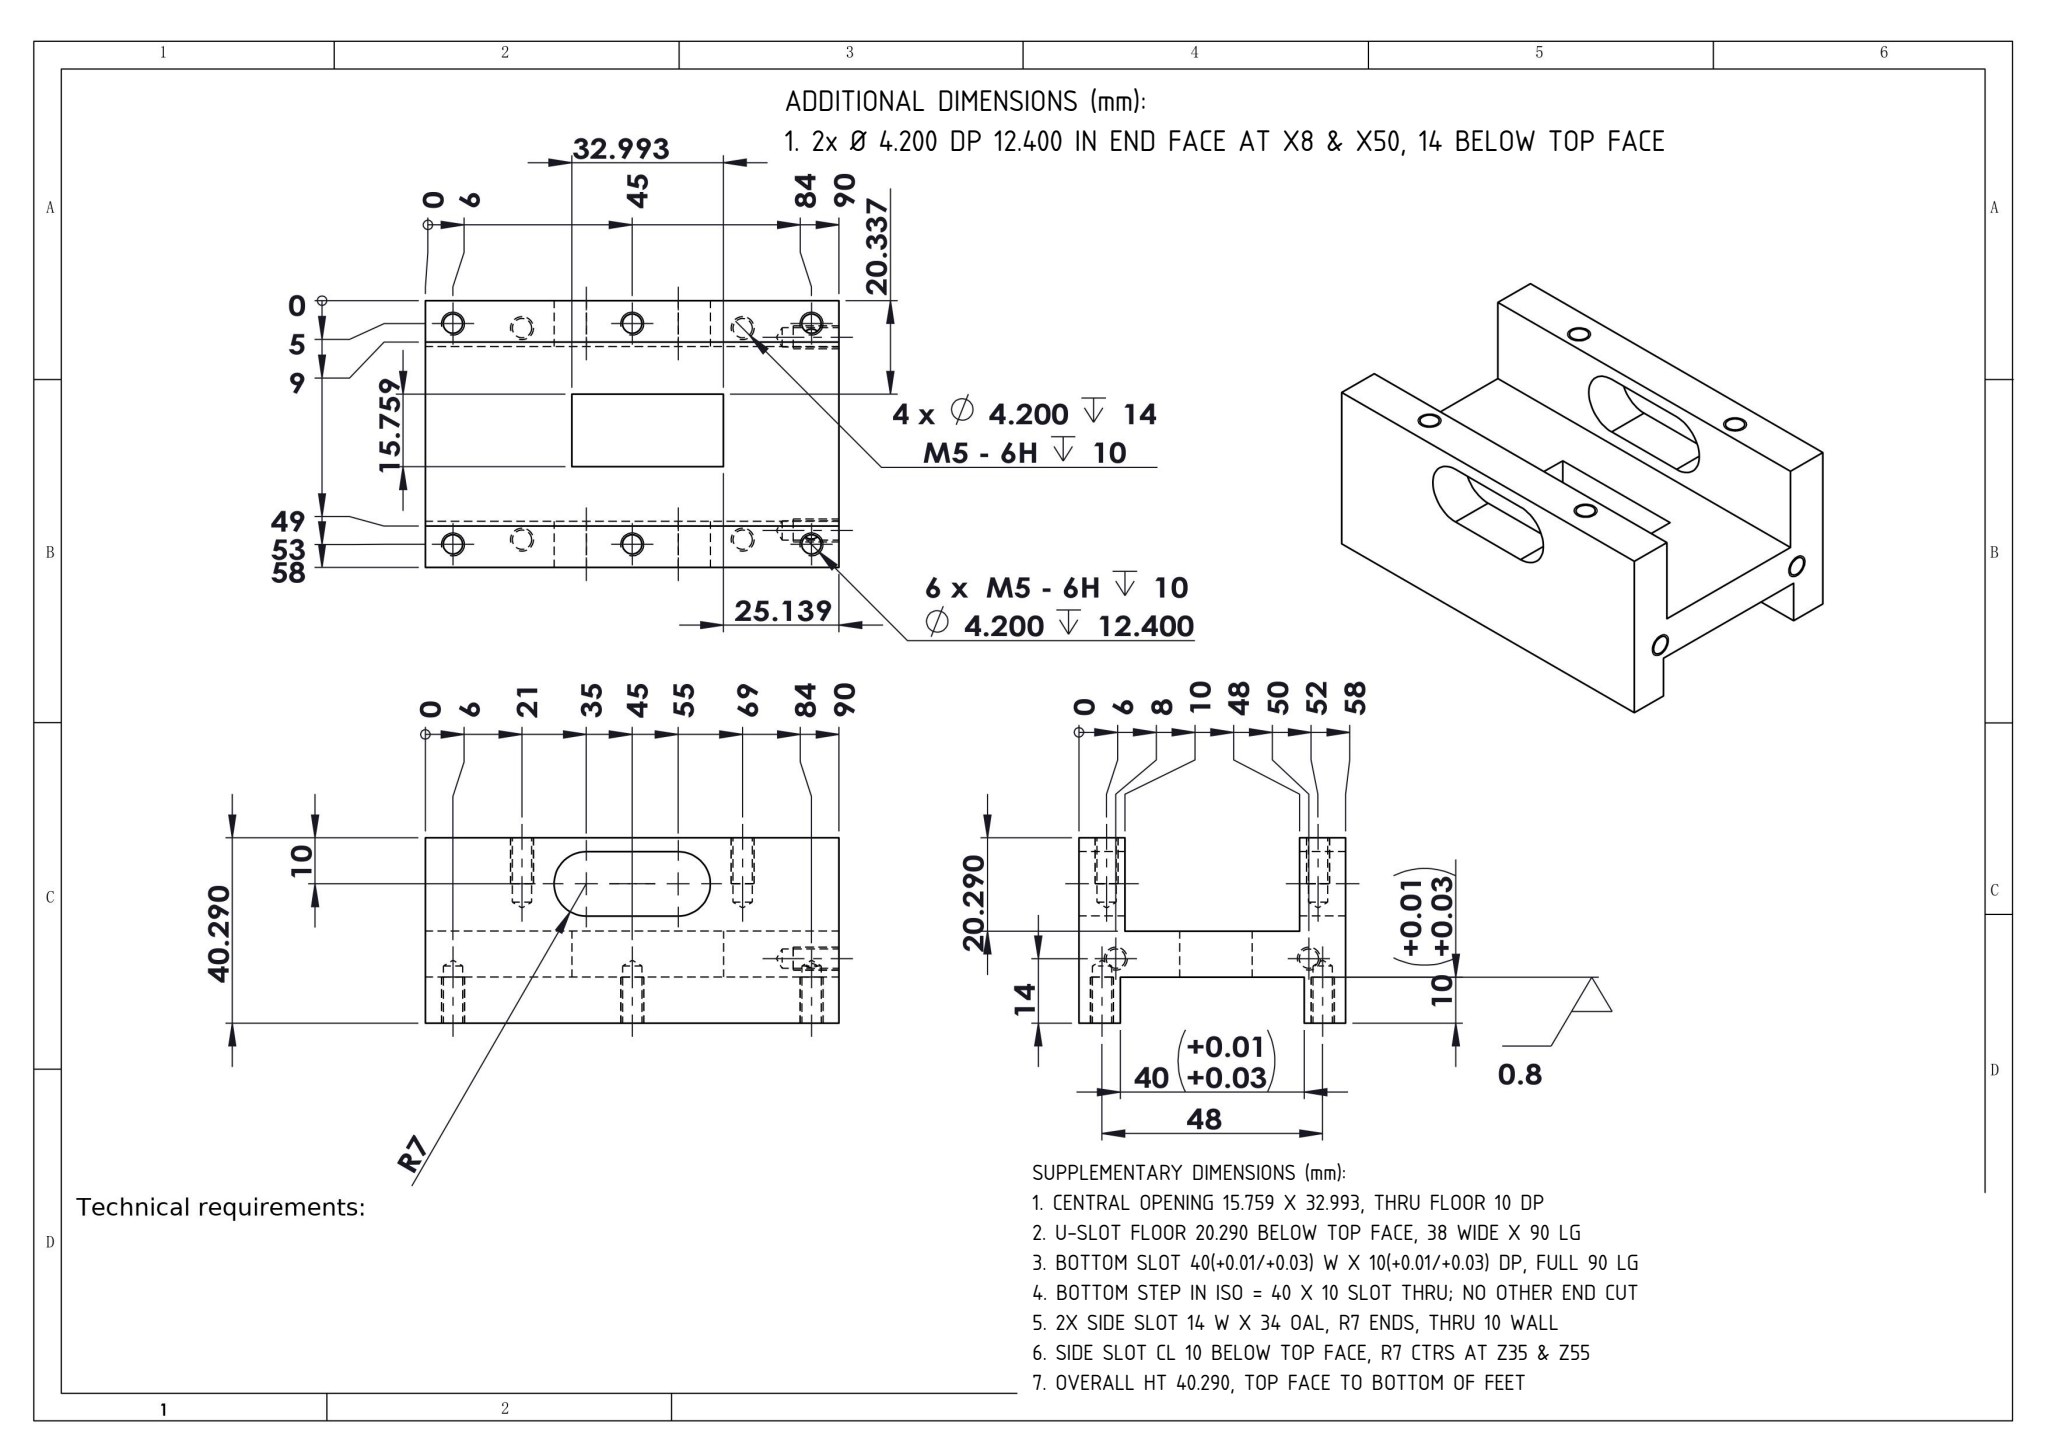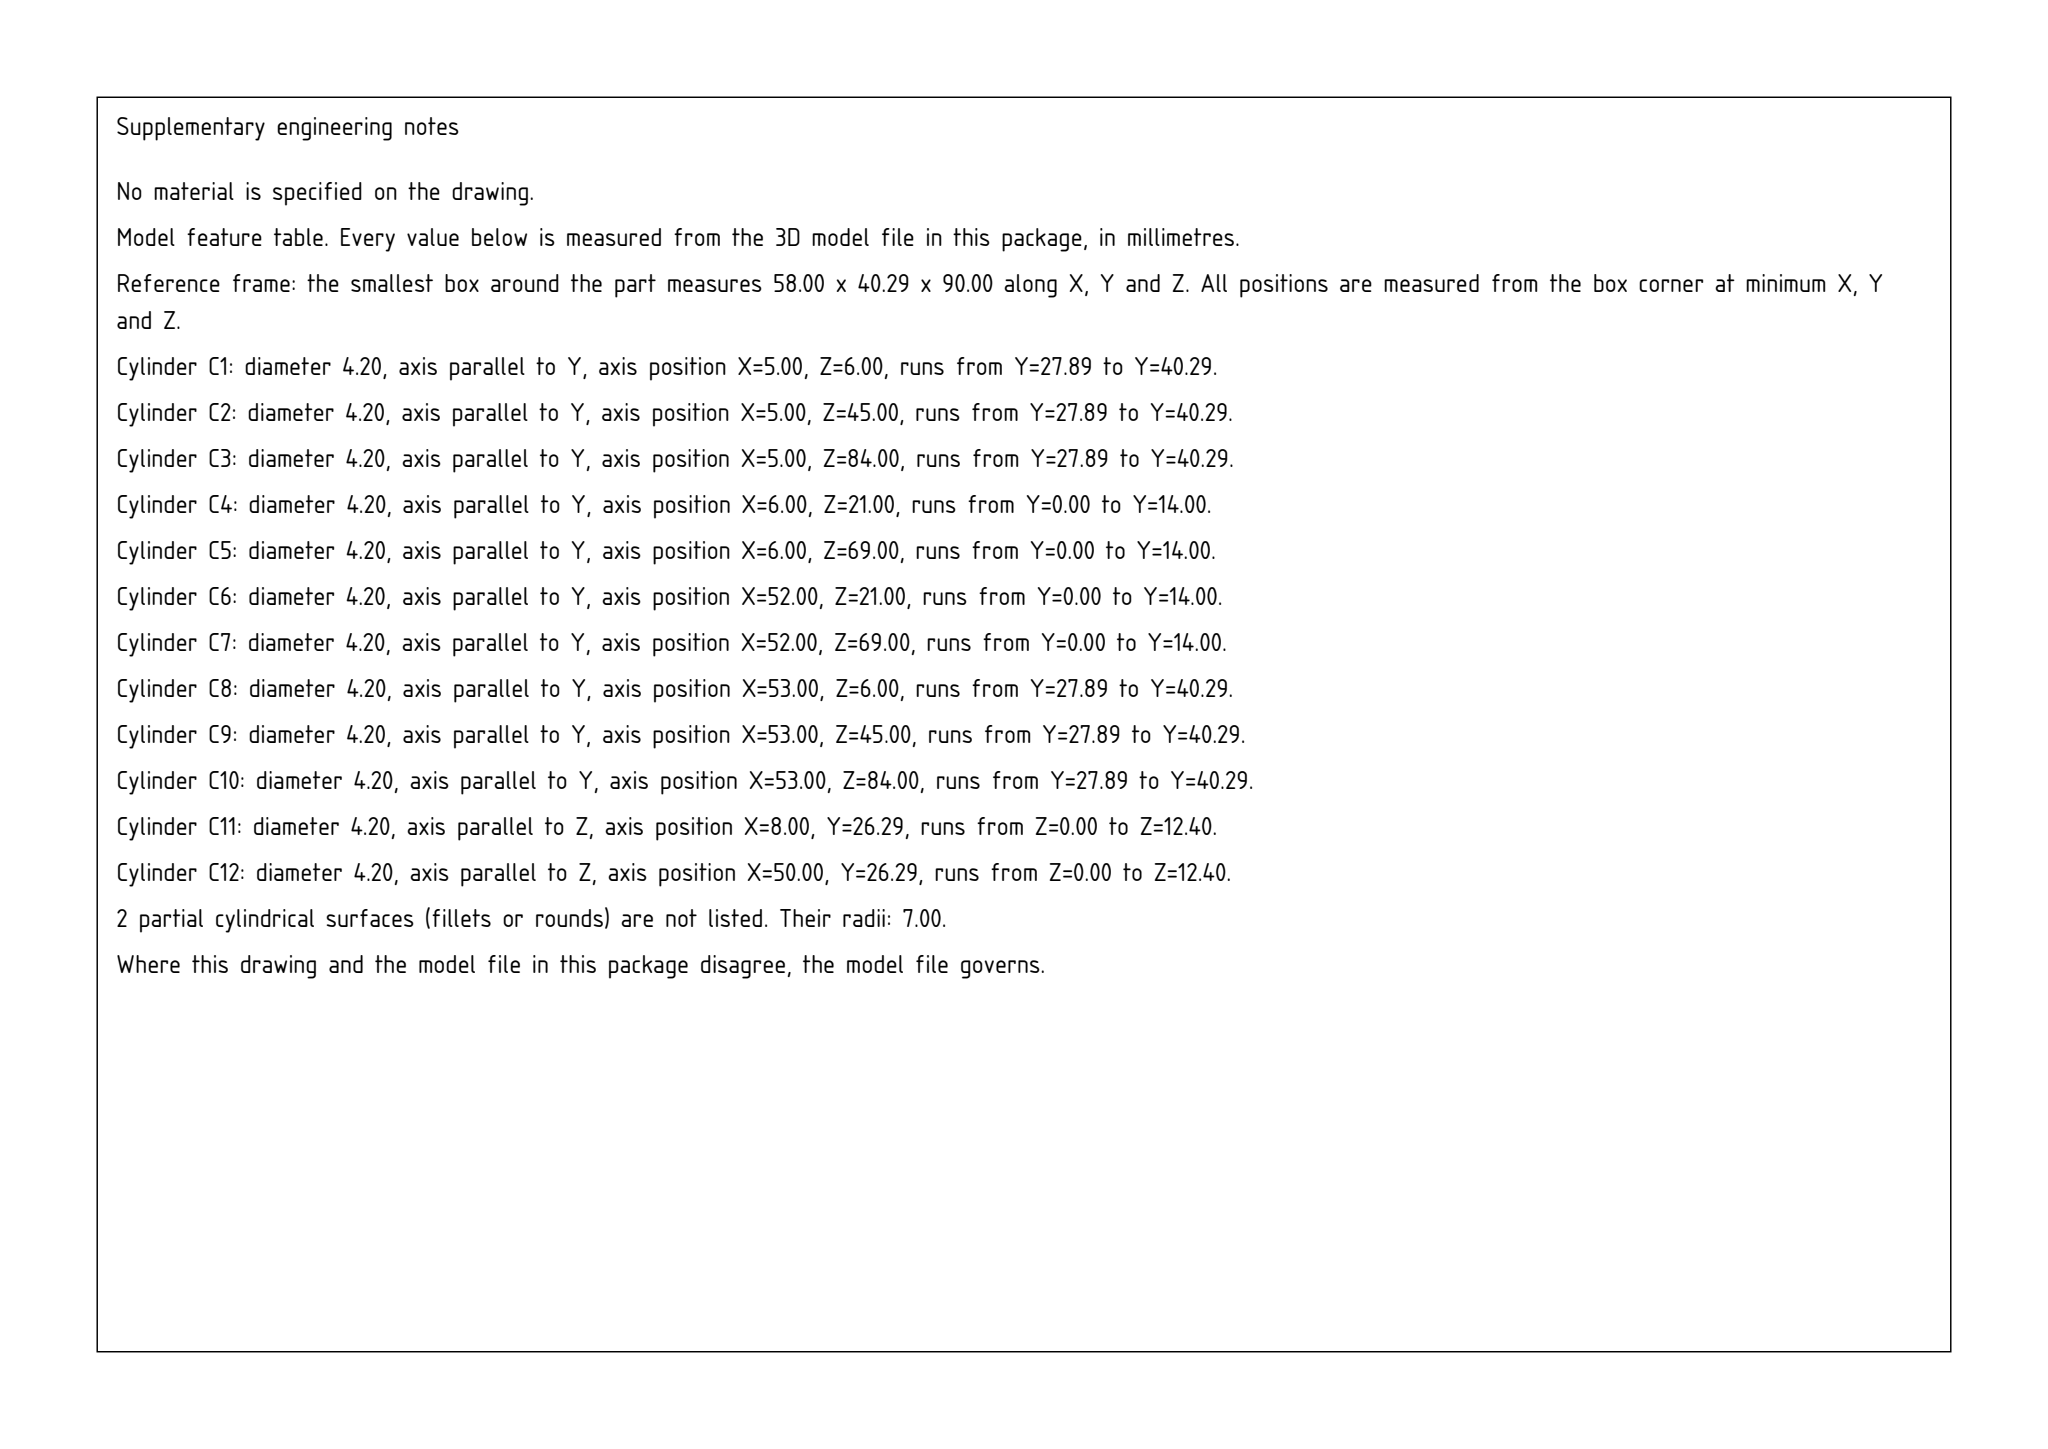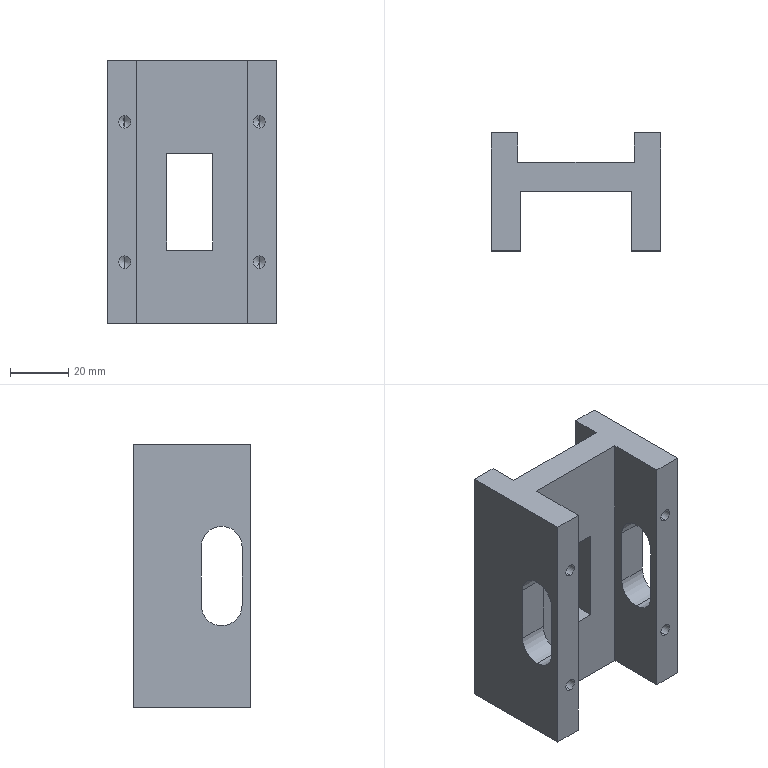Part | SolidWorks | mm | 1 solid | 76 faces | box 58 x 40.29 x 90 mm | volume 88824 mm3 | cylinder 30 | cone 24 | plane 22 | commonest cylinder face diameters 4.2 x24 14 x6
build123d program:
from build123d import *

# Parameters (mm, degrees)
SKETCH1_W             = 58
SKETCH1_H             = 90
BOSS_EXTRUDE1_DEPTH   = 40.29
SKETCH2_W             = 40
SKETCH2_H             = 90
CUT_EXTRUDE1_DEPTH    = 10
M5_TAPPED_HOLE1_D     = 4.2
M5_TAPPED_HOLE1_DEPTH = 14
M5_TAPPED_HOLE1_TIP   = 1.262
SKETCH5_W             = 38
SKETCH5_H             = 90
CUT_EXTRUDE2_DEPTH    = 20.29
M5_TAPPED_HOLE2_D     = 4.2
M5_TAPPED_HOLE2_DEPTH = 12.4
M5_TAPPED_HOLE2_TIP   = 1.262
M5_TAPPED_HOLE3_D     = 4.2
M5_TAPPED_HOLE3_DEPTH = 12.4
M5_TAPPED_HOLE3_TIP   = 1.262
CUT_EXTRUDE3_DEPTH    = 117
SKETCH11_W            = 15.759
SKETCH11_H            = 32.993
CUT_EXTRUDE4_DEPTH    = 28


with BuildPart() as part:
    # Sketch1 → Boss-Extrude1 (new body)
    with BuildSketch(Plane(origin=(0, 0, 0), x_dir=(1, 0, 0), z_dir=(0, 1, 0))):
        with Locations((29, 45)):
            Rectangle(SKETCH1_W, SKETCH1_H)
    extrude(amount=BOSS_EXTRUDE1_DEPTH)

    # Sketch2 → Cut-Extrude1 (cut)
    with BuildSketch(Plane(origin=(0, 40.29, 0), x_dir=(1, 0, 0), z_dir=(0, 1, 0))):
        with Locations((29, 45)):
            Rectangle(SKETCH2_W, SKETCH2_H)
    extrude(amount=-CUT_EXTRUDE1_DEPTH, mode=Mode.SUBTRACT)

    # M5 Tapped Hole1
    with Locations(Plane.XZ):
        with Locations((6, -21), (6, -69), (52, -69), (52, -21)):
            Hole(M5_TAPPED_HOLE1_D / 2, depth=M5_TAPPED_HOLE1_DEPTH)
            with Locations((0, 0, -(M5_TAPPED_HOLE1_DEPTH + M5_TAPPED_HOLE1_TIP / 2))):  # 118° drill point
                Cone(0, M5_TAPPED_HOLE1_D / 2, M5_TAPPED_HOLE1_TIP, mode=Mode.SUBTRACT)

    # Sketch5 → Cut-Extrude2 (cut)
    with BuildSketch(Plane.XZ):
        with Locations((29, -45)):
            Rectangle(SKETCH5_W, SKETCH5_H)
    extrude(amount=-CUT_EXTRUDE2_DEPTH, mode=Mode.SUBTRACT)

    # M5 Tapped Hole2
    with Locations(Plane(origin=(0, 40.29, 0), x_dir=(-1, 0, 0), z_dir=(0, 1, 0))):
        with Locations((-53, -84), (-53, -45), (-53, -6), (-5, -6), (-5, -45), (-5, -84)):
            Hole(M5_TAPPED_HOLE2_D / 2, depth=M5_TAPPED_HOLE2_DEPTH)
            with Locations((0, 0, -(M5_TAPPED_HOLE2_DEPTH + M5_TAPPED_HOLE2_TIP / 2))):  # 118° drill point
                Cone(0, M5_TAPPED_HOLE2_D / 2, M5_TAPPED_HOLE2_TIP, mode=Mode.SUBTRACT)

    # M5 Tapped Hole3
    with Locations(Plane(origin=(0, 0, -90), x_dir=(-1, 0, 0), z_dir=(0, 0, -1))):
        with Locations((-8, 26.29), (-50, 26.29)):
            Hole(M5_TAPPED_HOLE3_D / 2, depth=M5_TAPPED_HOLE3_DEPTH)
            with Locations((0, 0, -(M5_TAPPED_HOLE3_DEPTH + M5_TAPPED_HOLE3_TIP / 2))):  # 118° drill point
                Cone(0, M5_TAPPED_HOLE3_D / 2, M5_TAPPED_HOLE3_TIP, mode=Mode.SUBTRACT)

    # Sketch10 → Cut-Extrude3 (cut)
    with BuildSketch(Plane(origin=(58, 0, 0), x_dir=(0, 0, -1), z_dir=(1, 0, 0))):
        with BuildLine():
            Line((35, 17), (55, 17))
            ThreePointArc((55, 17), (62, 10), (55, 3))
            Line((55, 3), (35, 3))
            ThreePointArc((35, 3), (28, 10), (35, 17))
        make_face()
    extrude(amount=-CUT_EXTRUDE3_DEPTH, mode=Mode.SUBTRACT)

    # Sketch11 → Cut-Extrude4 (cut)
    with BuildSketch(Plane(origin=(0, 30.29, 0), x_dir=(1, 0, 0), z_dir=(0, 1, 0))):
        with Locations((28.217, 48.364)):
            Rectangle(SKETCH11_W, SKETCH11_H)
    extrude(amount=-CUT_EXTRUDE4_DEPTH, mode=Mode.SUBTRACT)


solid = part.part